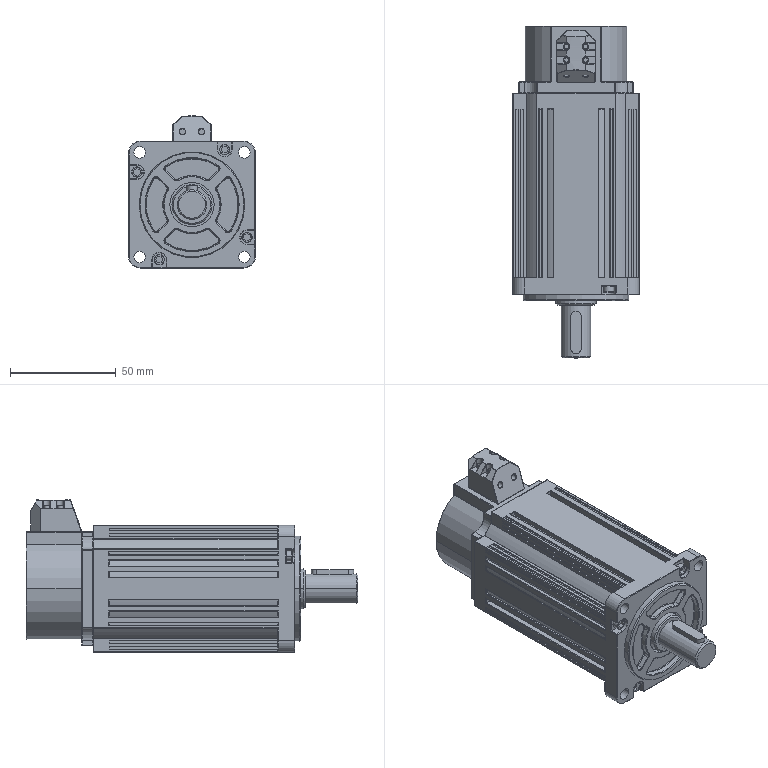Component | SolidWorks | 60-90SeriesServoMotor[60ST-M00630]_60ST-M00630-1 | 1 solid | 922 faces | volume 371769 mm3 | cylinder 358 | plane 344 | torus 137 | sphere 52 | spline 24 | cone 7 | commonest cylinder face diameters 0.4 x216 3 x20 0.6 x16 60 x16 2.54 x8 3.6 x8 3.78 x8 4.95 x8